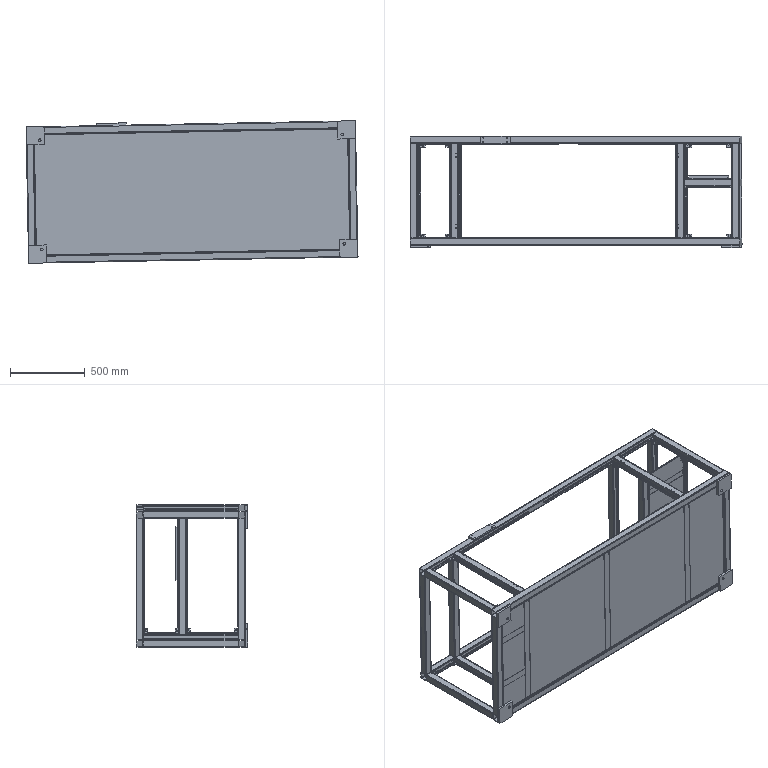Component | SolidWorks | 01Frame-1 | 81 solids | 1522 faces | volume 22885624 mm3 | plane 962 | cylinder 560 | commonest cylinder face diameters 6 x116 10 x88 4 x88 5 x56 2 x36 6.8 x36 8 x32 4.2 x32 | material A3 Steel